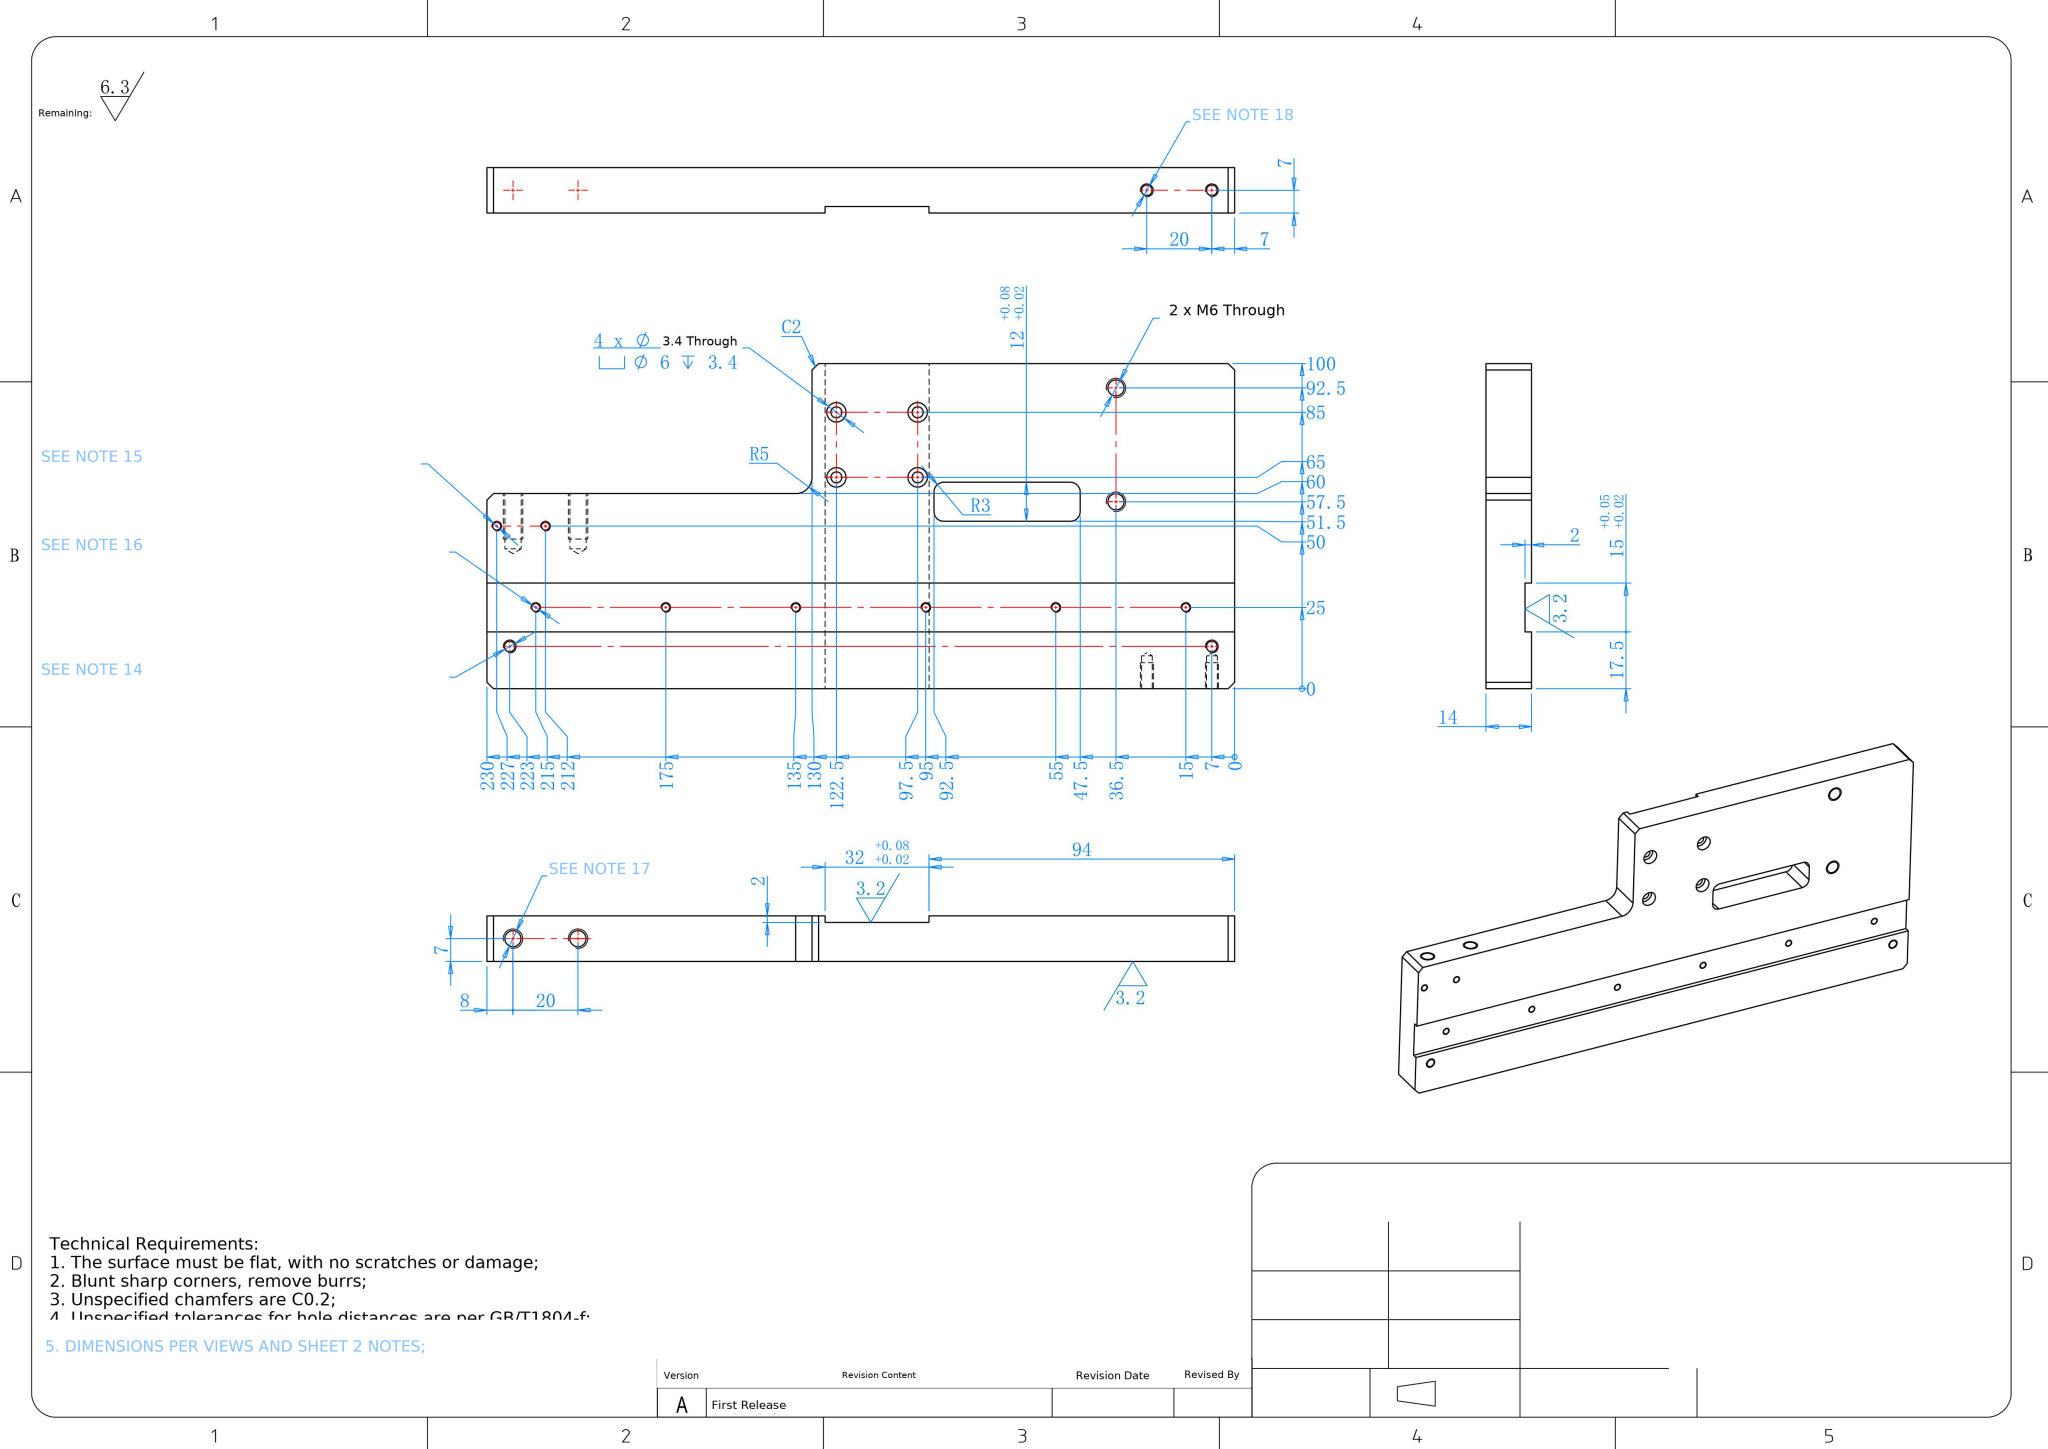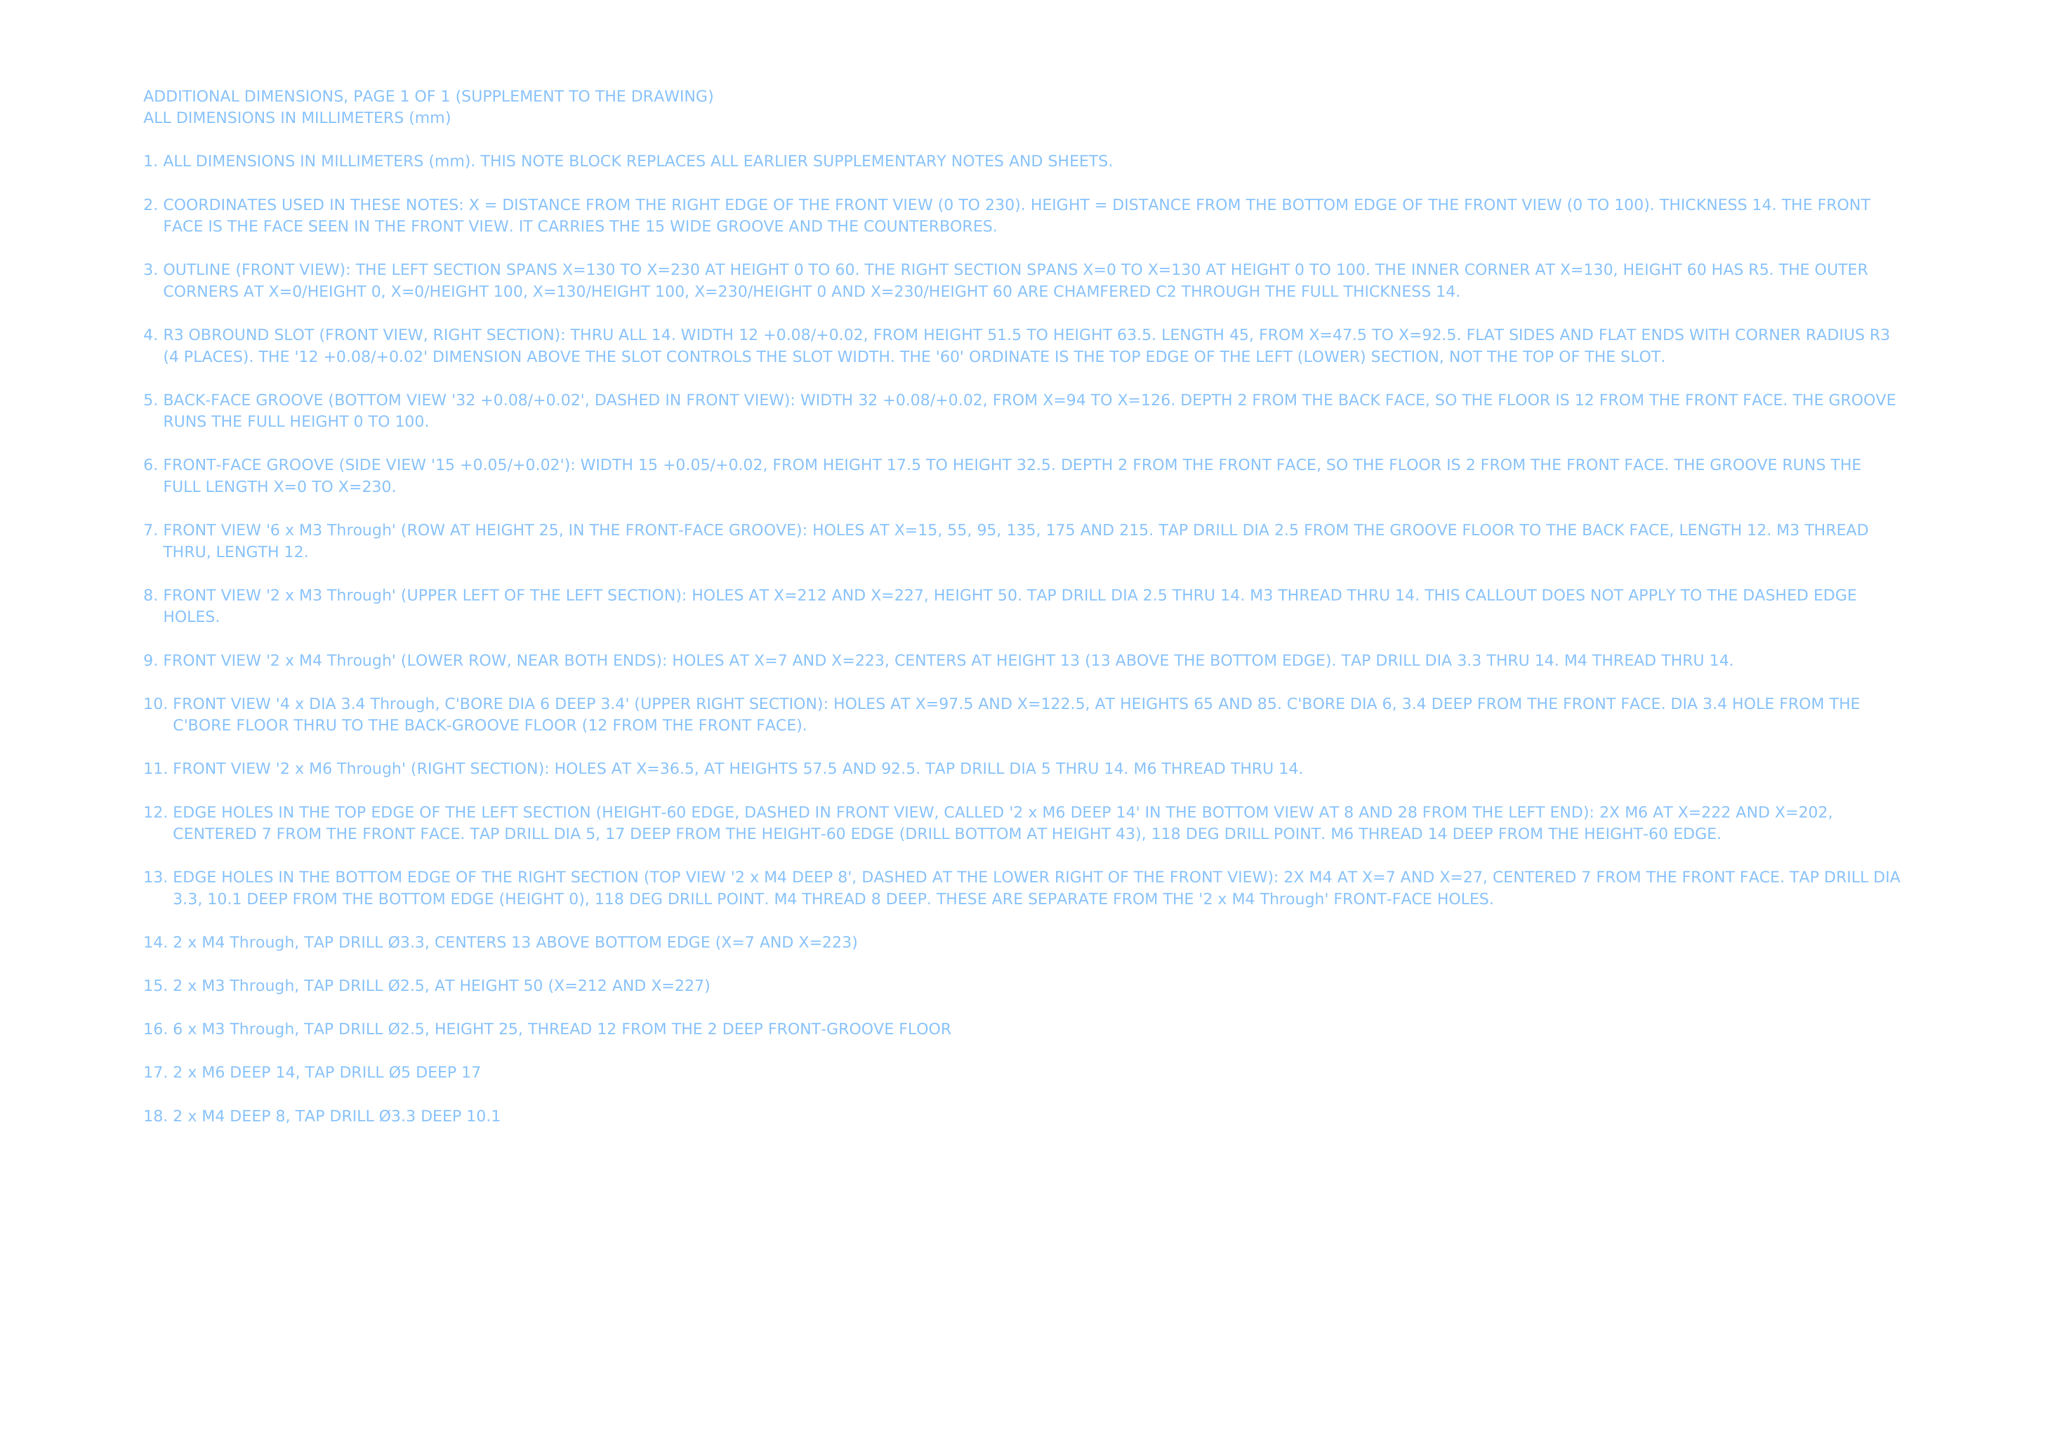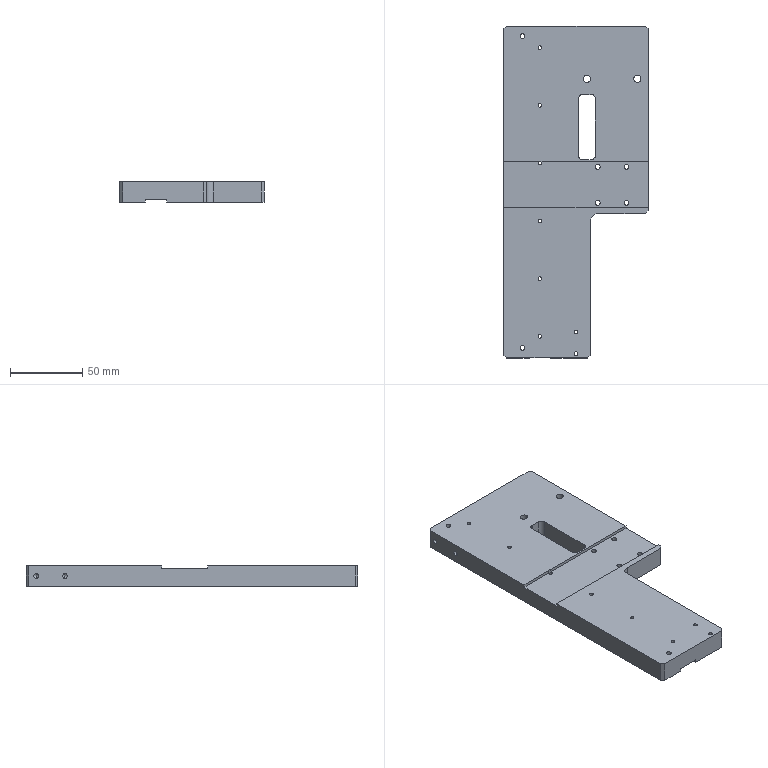Part | NX | mm | 1 solid | 91 faces | box 100 x 230 x 14 mm | volume 242350 mm3 | cylinder 53 | plane 30 | cone 8 | commonest cylinder face diameters 2.5 x16 6 x12 3.3 x8 5 x8 3.4 x8 10 x1